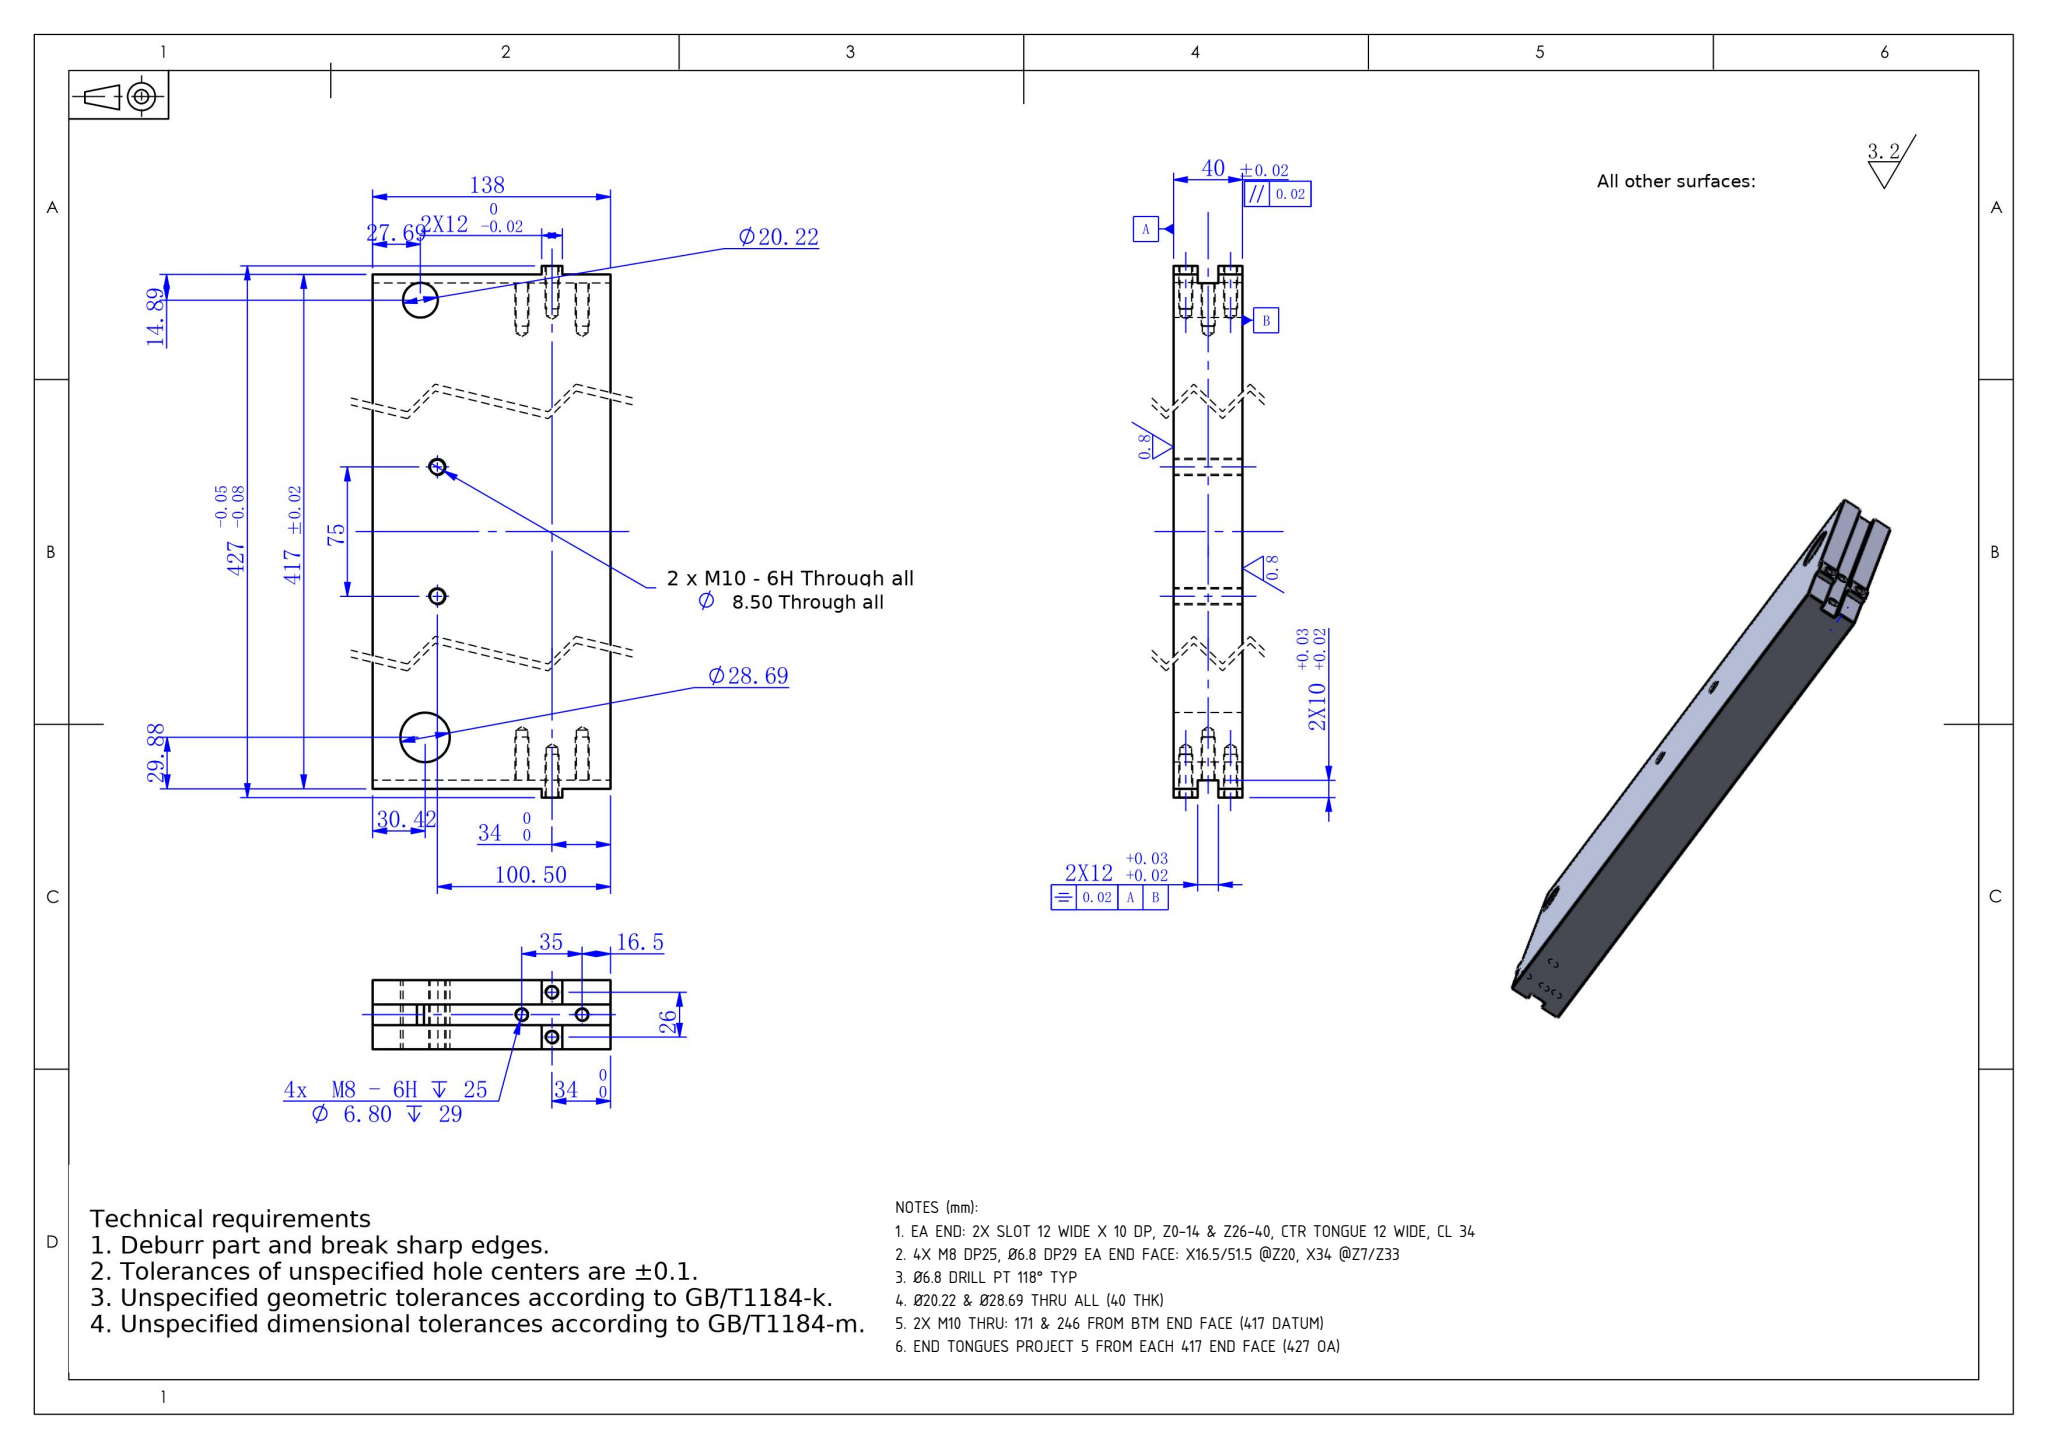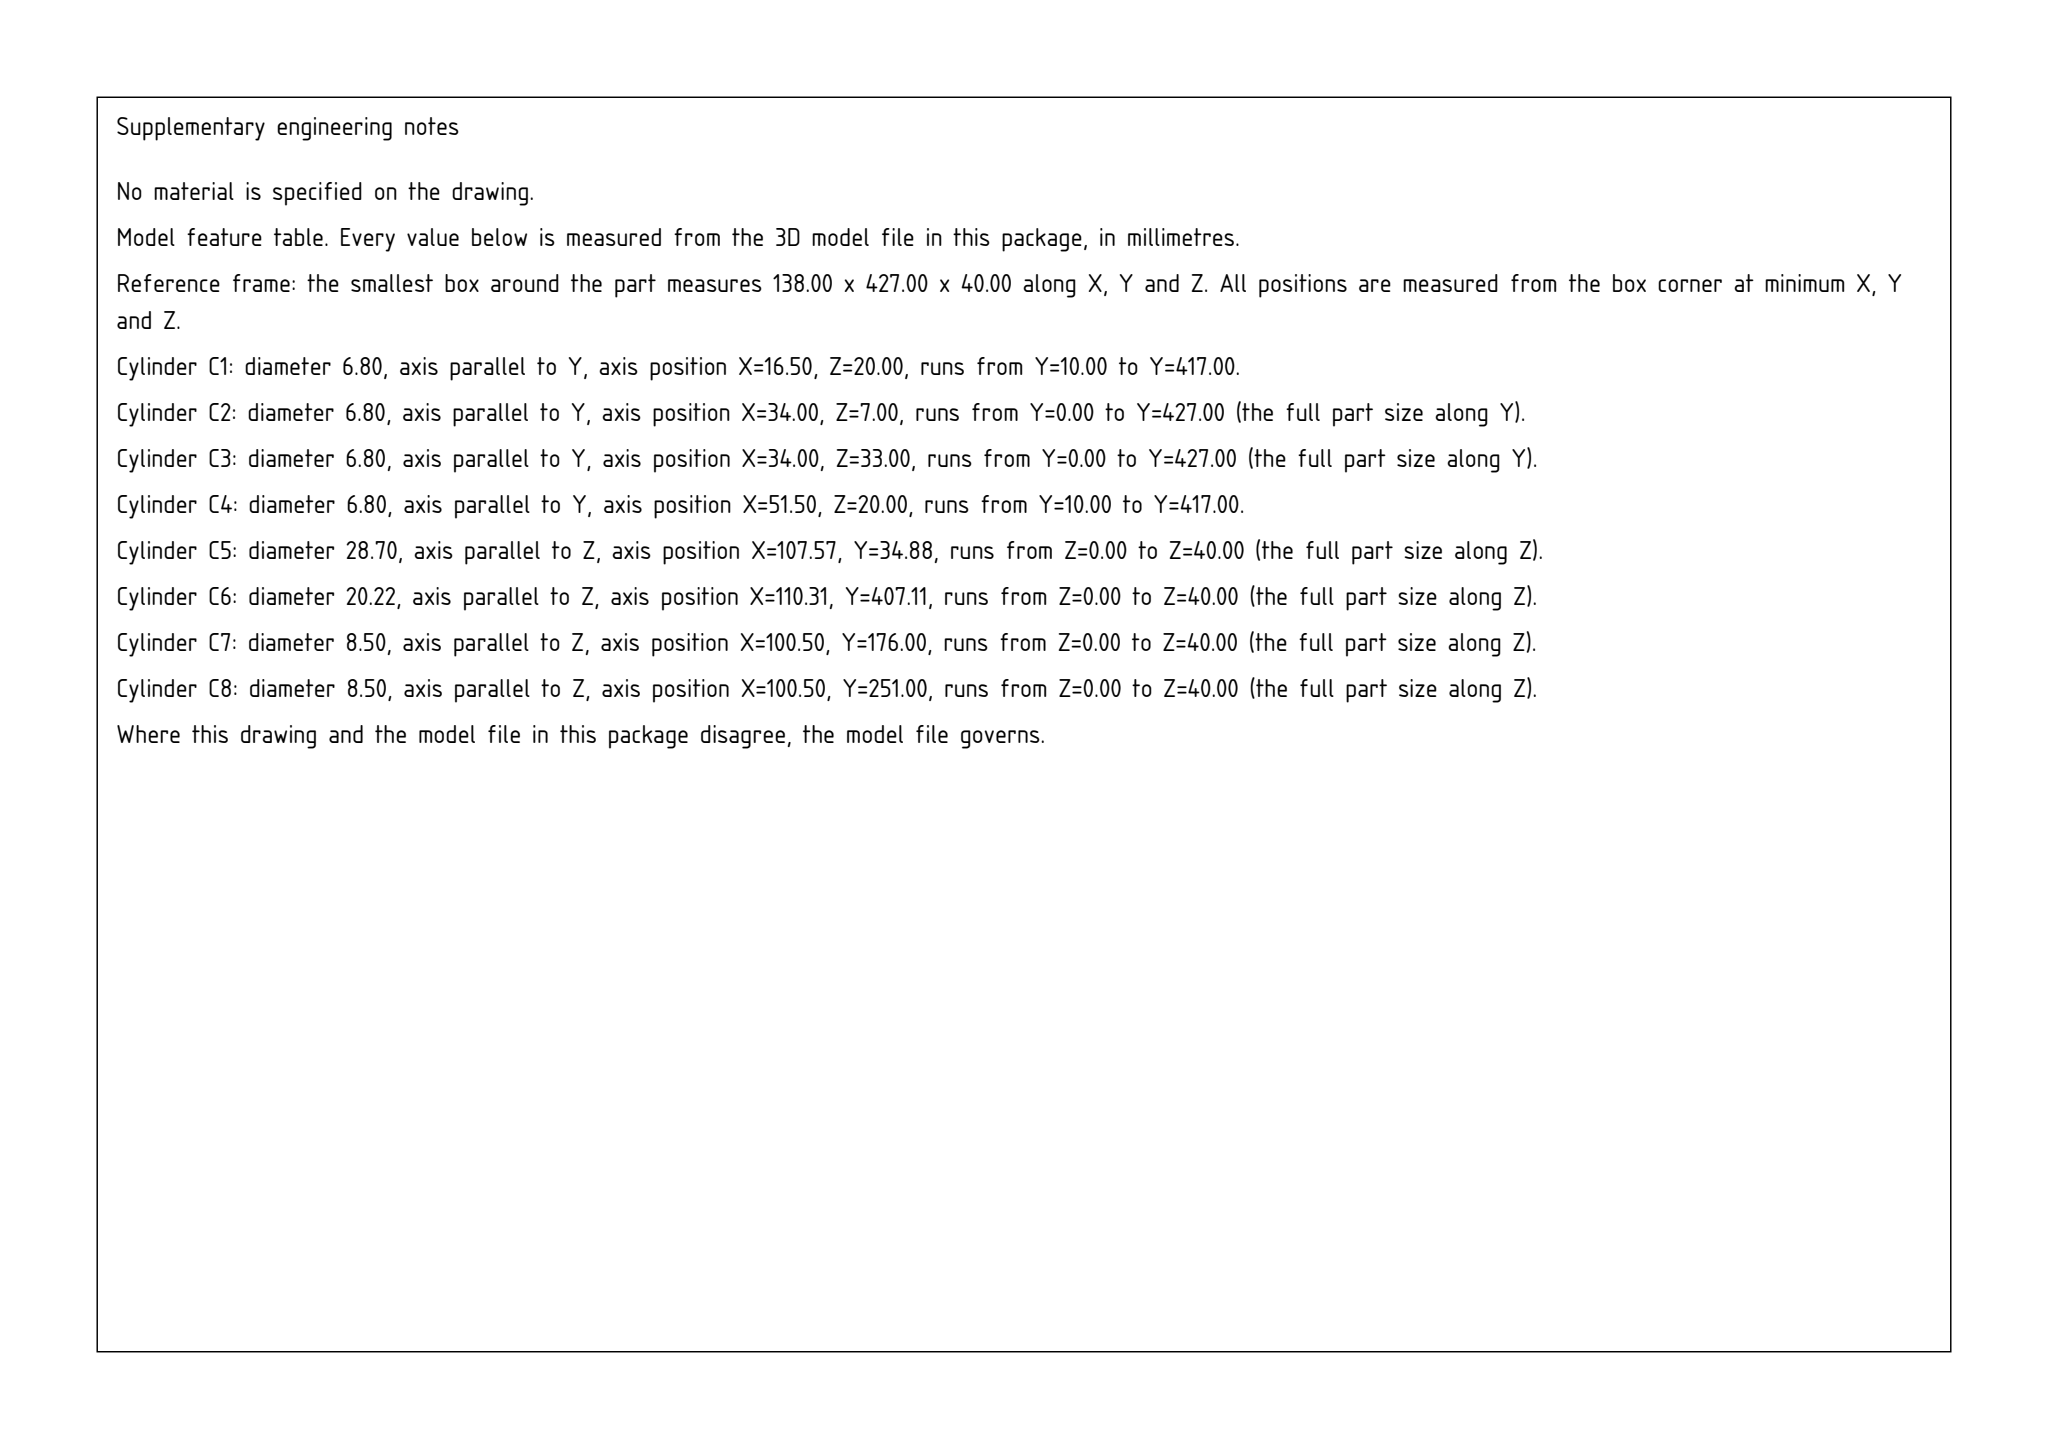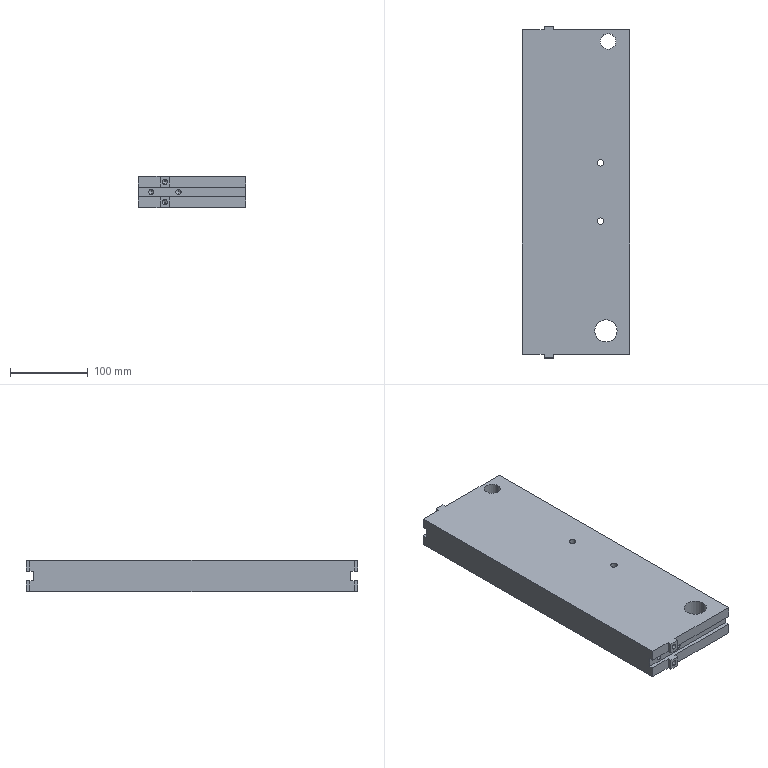Part | SolidWorks | mm | 1 solid | 71 faces | box 138 x 427 x 40 mm | volume 2236775 mm3 | plane 31 | cylinder 24 | cone 16 | commonest cylinder face diameters 6.8 x16 8.5 x4 28.694 x2 20.22 x2
Drawing notes:
EA END: 2X SLOT 12 WIDE X 10 DP, Z0-14 & Z26-40, CTR TONGUE 12 WIDE, CL 34 | from the solid: x planes 28 & 40 = 12 wide slots, CL x=34; z planes 14 & 26 bound 12 wide tongue; slot floors y=10 / y=417 from end faces y=0 / y=427
4X M8 DP25, Ø6.8 DP29 EA END FACE: X16.5/51.5 @Z20, X34 @Z7/Z33 | from the solid: Ø6.8 cyls axis y, len 29 at (16.5,20),(51.5,20),(34,7),(34,33); pattern on both y=0 and y=427 end faces
Ø6.8 DRILL PT 118° TYP | from the solid: cones[included_angle,ref_dia] = 118°, ref dia 6.8
Ø20.22 & Ø28.69 THRU ALL (40 THK) | from the solid: cyls dia 20.22 and 28.694, axis z, length 40 = full bbox z (z planes 0 and 40)
2X M10 THRU: 171 & 246 FROM BTM END FACE (417 DATUM) | from the solid: Ø8.50 z-axis holes at y=176.0 and y=251.0; lower 417 end face plane y=5.0 -> 171 and 246; symmetric about 417 midplane y=213.5
END TONGUES PROJECT 5 FROM EACH 417 END FACE (427 OA) | from the solid: axis planes y=0 & y=427 (tongue tips) vs y=5.0 & y=422.0 (end faces); 422-5=417, 427-0=427, step=5 each end
build123d program:
from build123d import *

# Parameters (mm, degrees)
SKETCH1_W                  = 138
SKETCH1_H                  = 417
BOSS_EXTRUDE1_DEPTH        = 40
SKETCH2_W                  = 12
SKETCH2_H                  = 5
CUT_EXTRUDE1_DEPTH         = 2676.183
SKETCH4_W                  = 12
SKETCH4_H                  = 10
BOSS_EXTRUDE2_DEPTH        = 40
SKETCH5_W                  = 12
SKETCH5_H                  = 10
CUT_EXTRUDE2_DEPTH         = 2679.857
M8_TAPPED_HOLE1_AT_2_COUNT = 2
M8_TAPPED_HOLE1_AT_2_PITCH = 26
M8_TAPPED_HOLE2_AT_2_COUNT = 2
M8_TAPPED_HOLE2_AT_2_PITCH = 35
M10_TAPPED_HOLE1_D         = 8.5
SKETCH12_R                 = 14.347
SKETCH12_R_2               = 10.11
CUT_EXTRUDE4_DEPTH         = 107


with BuildPart() as part:
    # Sketch1 → Boss-Extrude1 (new body)
    with BuildSketch(Plane.XY.offset(259.6)):
        with Locations((-3351.015, -2450.478)):
            Rectangle(SKETCH1_W, SKETCH1_H)
    extrude(amount=-BOSS_EXTRUDE1_DEPTH)

    # Sketch2 → Cut-Extrude1 (cut, through all)
    with BuildSketch(Plane(origin=(-3282.015, 0, 0), x_dir=(0, 0, -1), z_dir=(1, 0, 0))):
        with Locations((-239.6, -2656.478)):
            Rectangle(SKETCH2_W, SKETCH2_H)
        with Locations((-239.6, -2244.478)):
            Rectangle(SKETCH2_W, SKETCH2_H)
    cut_extrude1 = extrude(amount=-CUT_EXTRUDE1_DEPTH, mode=Mode.SUBTRACT)

    # Sketch4 → Boss-Extrude2 (add, through all)
    with BuildSketch(Plane.XY.offset(259.6)):
        with Locations((-3386.015, -2658.978)):
            Rectangle(SKETCH4_W, SKETCH4_H)
    boss_extrude2 = extrude(amount=-BOSS_EXTRUDE2_DEPTH)

    # Sketch5 → Cut-Extrude2 (cut, through all)
    with BuildSketch(Plane.ZY.offset(3392.015)):
        with Locations((239.6, -2658.978)):
            Rectangle(SKETCH5_W, SKETCH5_H)
    cut_extrude2 = extrude(amount=-CUT_EXTRUDE2_DEPTH, mode=Mode.SUBTRACT)

    # Sketch6 → M8 Tapped Hole1 (revolve, cut)
    with BuildSketch(Plane(origin=(-3386.015, -2663.978, 252.6), x_dir=(0, 0, -1), z_dir=(1, 0, 0))):
        Polygon((0, 0), (0, 31.043), (3.4, 29), (3.4, 0), align=None)
    m8_tapped_hole1 = revolve(axis=Axis((-3386.015, -2670.328, 252.6), (0, 1, 0)), mode=Mode.SUBTRACT)

    # M8 Tapped Hole1 at 2: M8 Tapped Hole1 ×2
    with Locations(*[(0, 0, -i * M8_TAPPED_HOLE1_AT_2_PITCH) for i in range(1, M8_TAPPED_HOLE1_AT_2_COUNT)]):
        add(m8_tapped_hole1, mode=Mode.SUBTRACT)

    # Sketch8 → M8 Tapped Hole2 (revolve, cut)
    with BuildSketch(Plane(origin=(-3403.515, -2653.978, 239.6), x_dir=(0, 0, -1), z_dir=(1, 0, 0))):
        Polygon((0, 0), (0, 31.043), (3.4, 29), (3.4, 0), align=None)
    m8_tapped_hole2 = revolve(axis=Axis((-3403.515, -2660.328, 239.6), (0, 1, 0)), mode=Mode.SUBTRACT)

    # M8 Tapped Hole2 at 2: M8 Tapped Hole2 ×2
    with Locations(*[(i * M8_TAPPED_HOLE2_AT_2_PITCH, 0, 0) for i in range(1, M8_TAPPED_HOLE2_AT_2_COUNT)]):
        add(m8_tapped_hole2, mode=Mode.SUBTRACT)

    # Mirror1: Cut-Extrude1, Boss-Extrude2, Cut-Extrude2, M8 Tapped Hole1, M8 Tapped Hole2 across plane
    add(cut_extrude1.mirror(Plane(origin=(0, -2450.478, 0), x_dir=(0, 0, 1), z_dir=(0, -1, 0))), mode=Mode.SUBTRACT)
    add(boss_extrude2.mirror(Plane(origin=(0, -2450.478, 0), x_dir=(0, 0, 1), z_dir=(0, -1, 0))))
    add(cut_extrude2.mirror(Plane(origin=(0, -2450.478, 0), x_dir=(0, 0, 1), z_dir=(0, -1, 0))), mode=Mode.SUBTRACT)
    add(m8_tapped_hole1.mirror(Plane(origin=(0, -2450.478, 0), x_dir=(0, 0, 1), z_dir=(0, -1, 0))), mode=Mode.SUBTRACT)
    add(m8_tapped_hole2.mirror(Plane(origin=(0, -2450.478, 0), x_dir=(0, 0, 1), z_dir=(0, -1, 0))), mode=Mode.SUBTRACT)

    # Mirror1 copy 1 sketch → Mirror1 copy 1 (revolve, cut)
    with BuildSketch(Plane(origin=(-3386.015, -2236.978, 226.6), x_dir=(0, 0, -1), z_dir=(1, 0, 0))):
        Polygon((0, 0), (0, -31.043), (3.4, -29), (3.4, 0), align=None)
    revolve(axis=Axis((-3386.015, -2230.628, 226.6), (0, 1, 0)), mode=Mode.SUBTRACT)

    # Mirror1 copy 2 sketch → Mirror1 copy 2 (revolve, cut)
    with BuildSketch(Plane(origin=(-3368.515, -2246.978, 239.6), x_dir=(0, 0, -1), z_dir=(1, 0, 0))):
        Polygon((0, 0), (0, -31.043), (3.4, -29), (3.4, 0), align=None)
    revolve(axis=Axis((-3368.515, -2240.628, 239.6), (0, 1, 0)), mode=Mode.SUBTRACT)

    # M10 Tapped Hole1 (through all)
    with Locations(Plane.XY.offset(259.6)):
        with Locations((-3319.515, -2487.978), (-3319.515, -2412.978)):
            Hole(M10_TAPPED_HOLE1_D / 2)

    # Sketch12 → Cut-Extrude4 (cut)
    with BuildSketch(Plane.XY.offset(259.6)):
        with Locations((-3312.437, -2629.103)):
            Circle(SKETCH12_R)
        with Locations((-3309.703, -2256.871)):
            Circle(SKETCH12_R_2)
    extrude(amount=-CUT_EXTRUDE4_DEPTH, mode=Mode.SUBTRACT)


solid = part.part